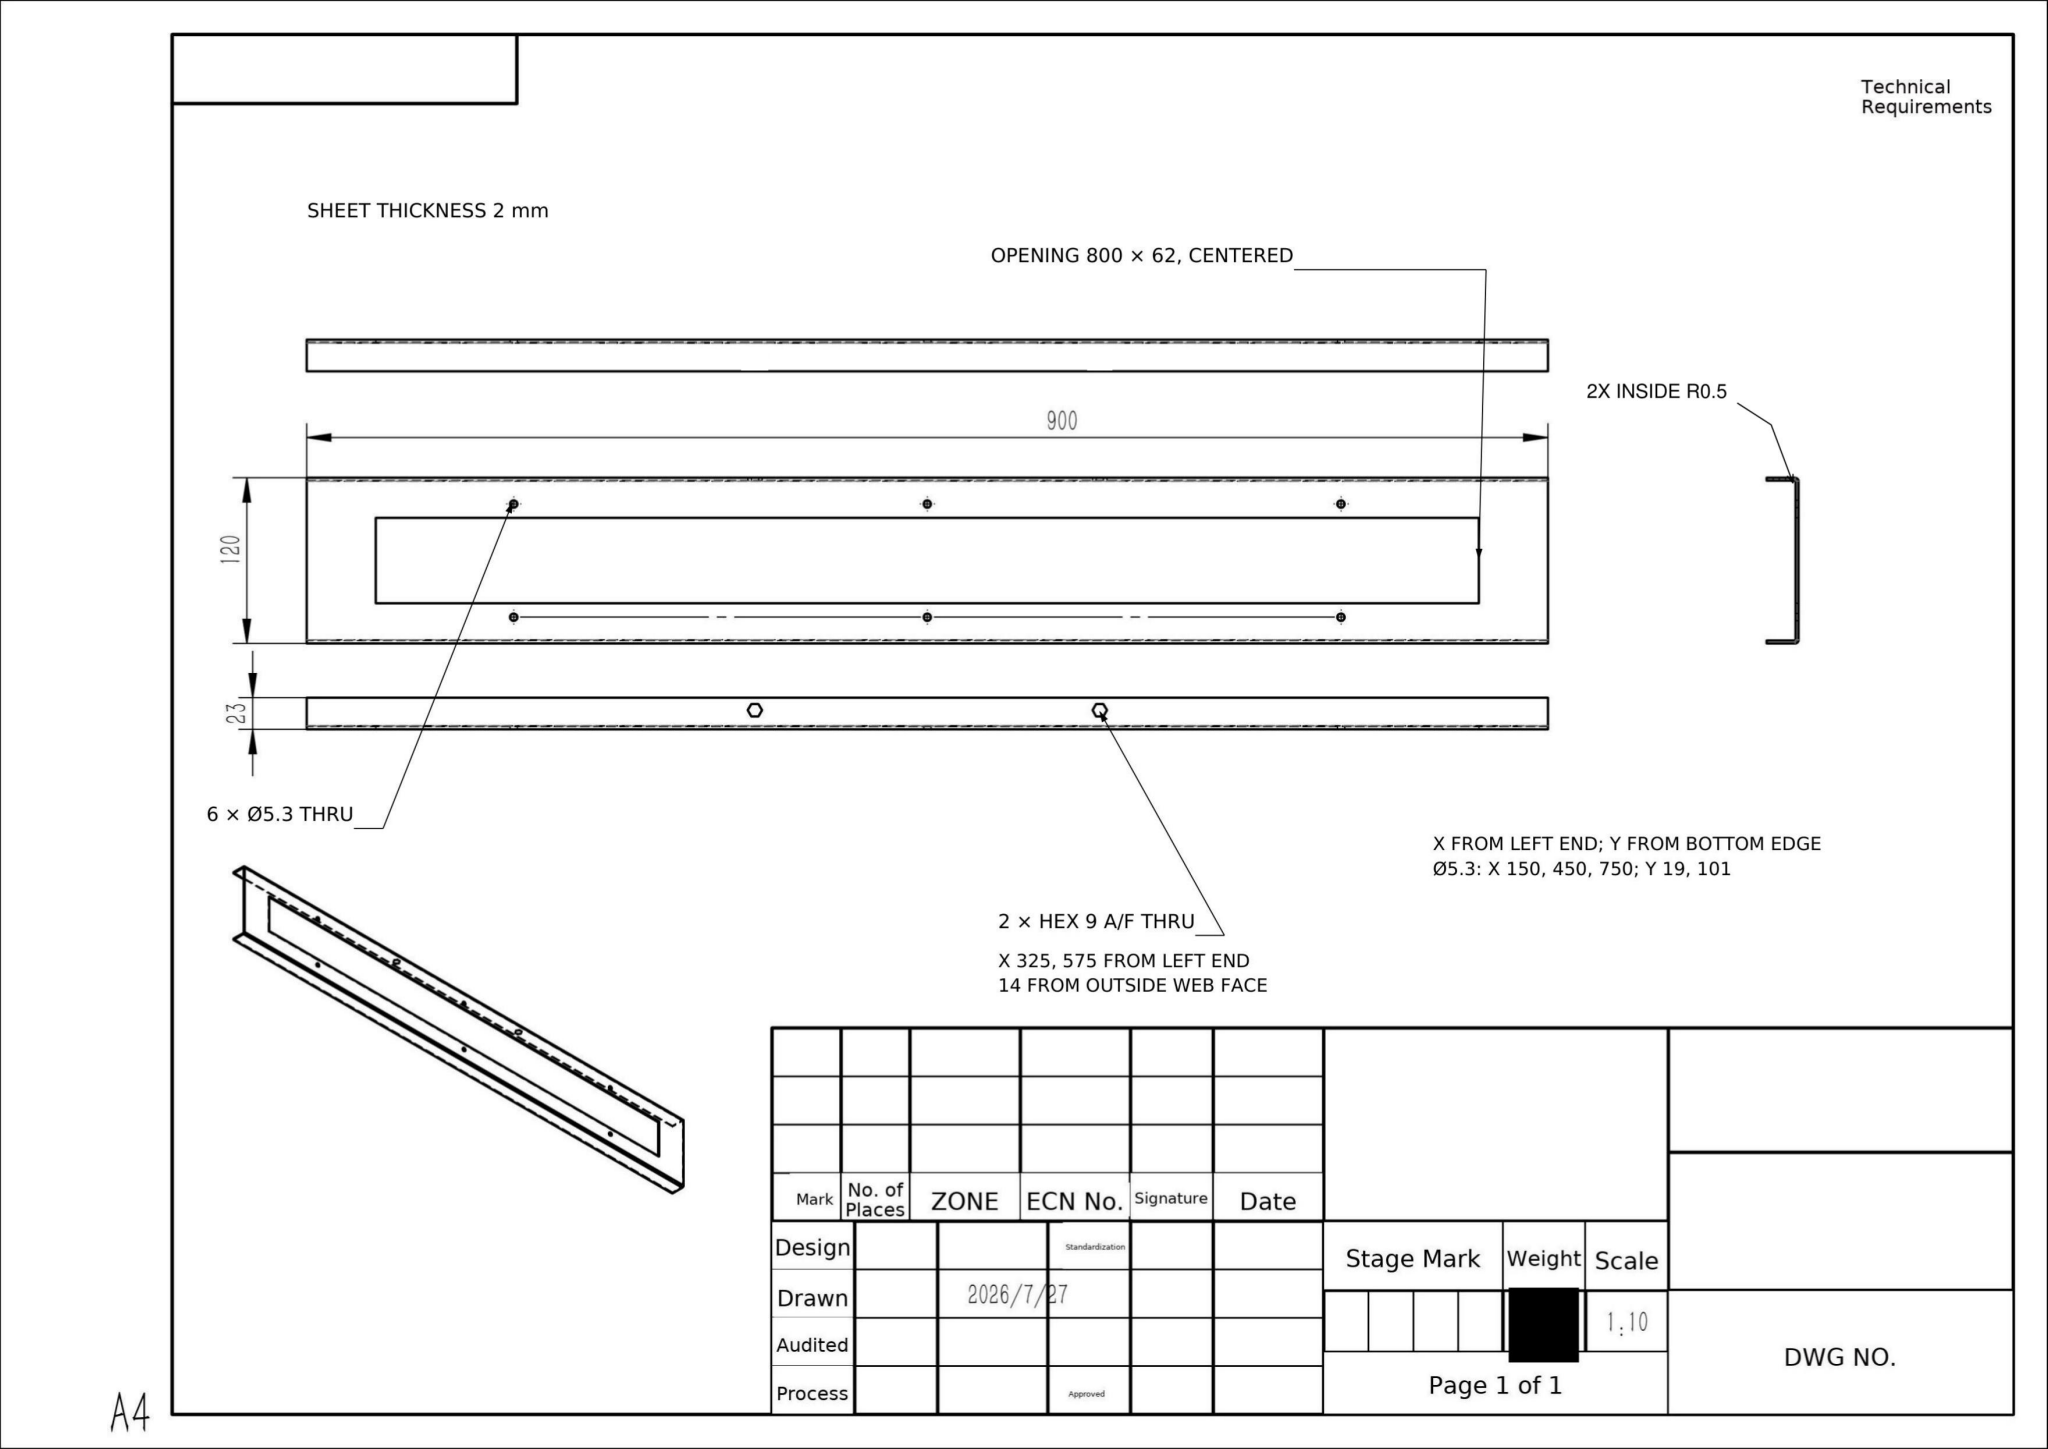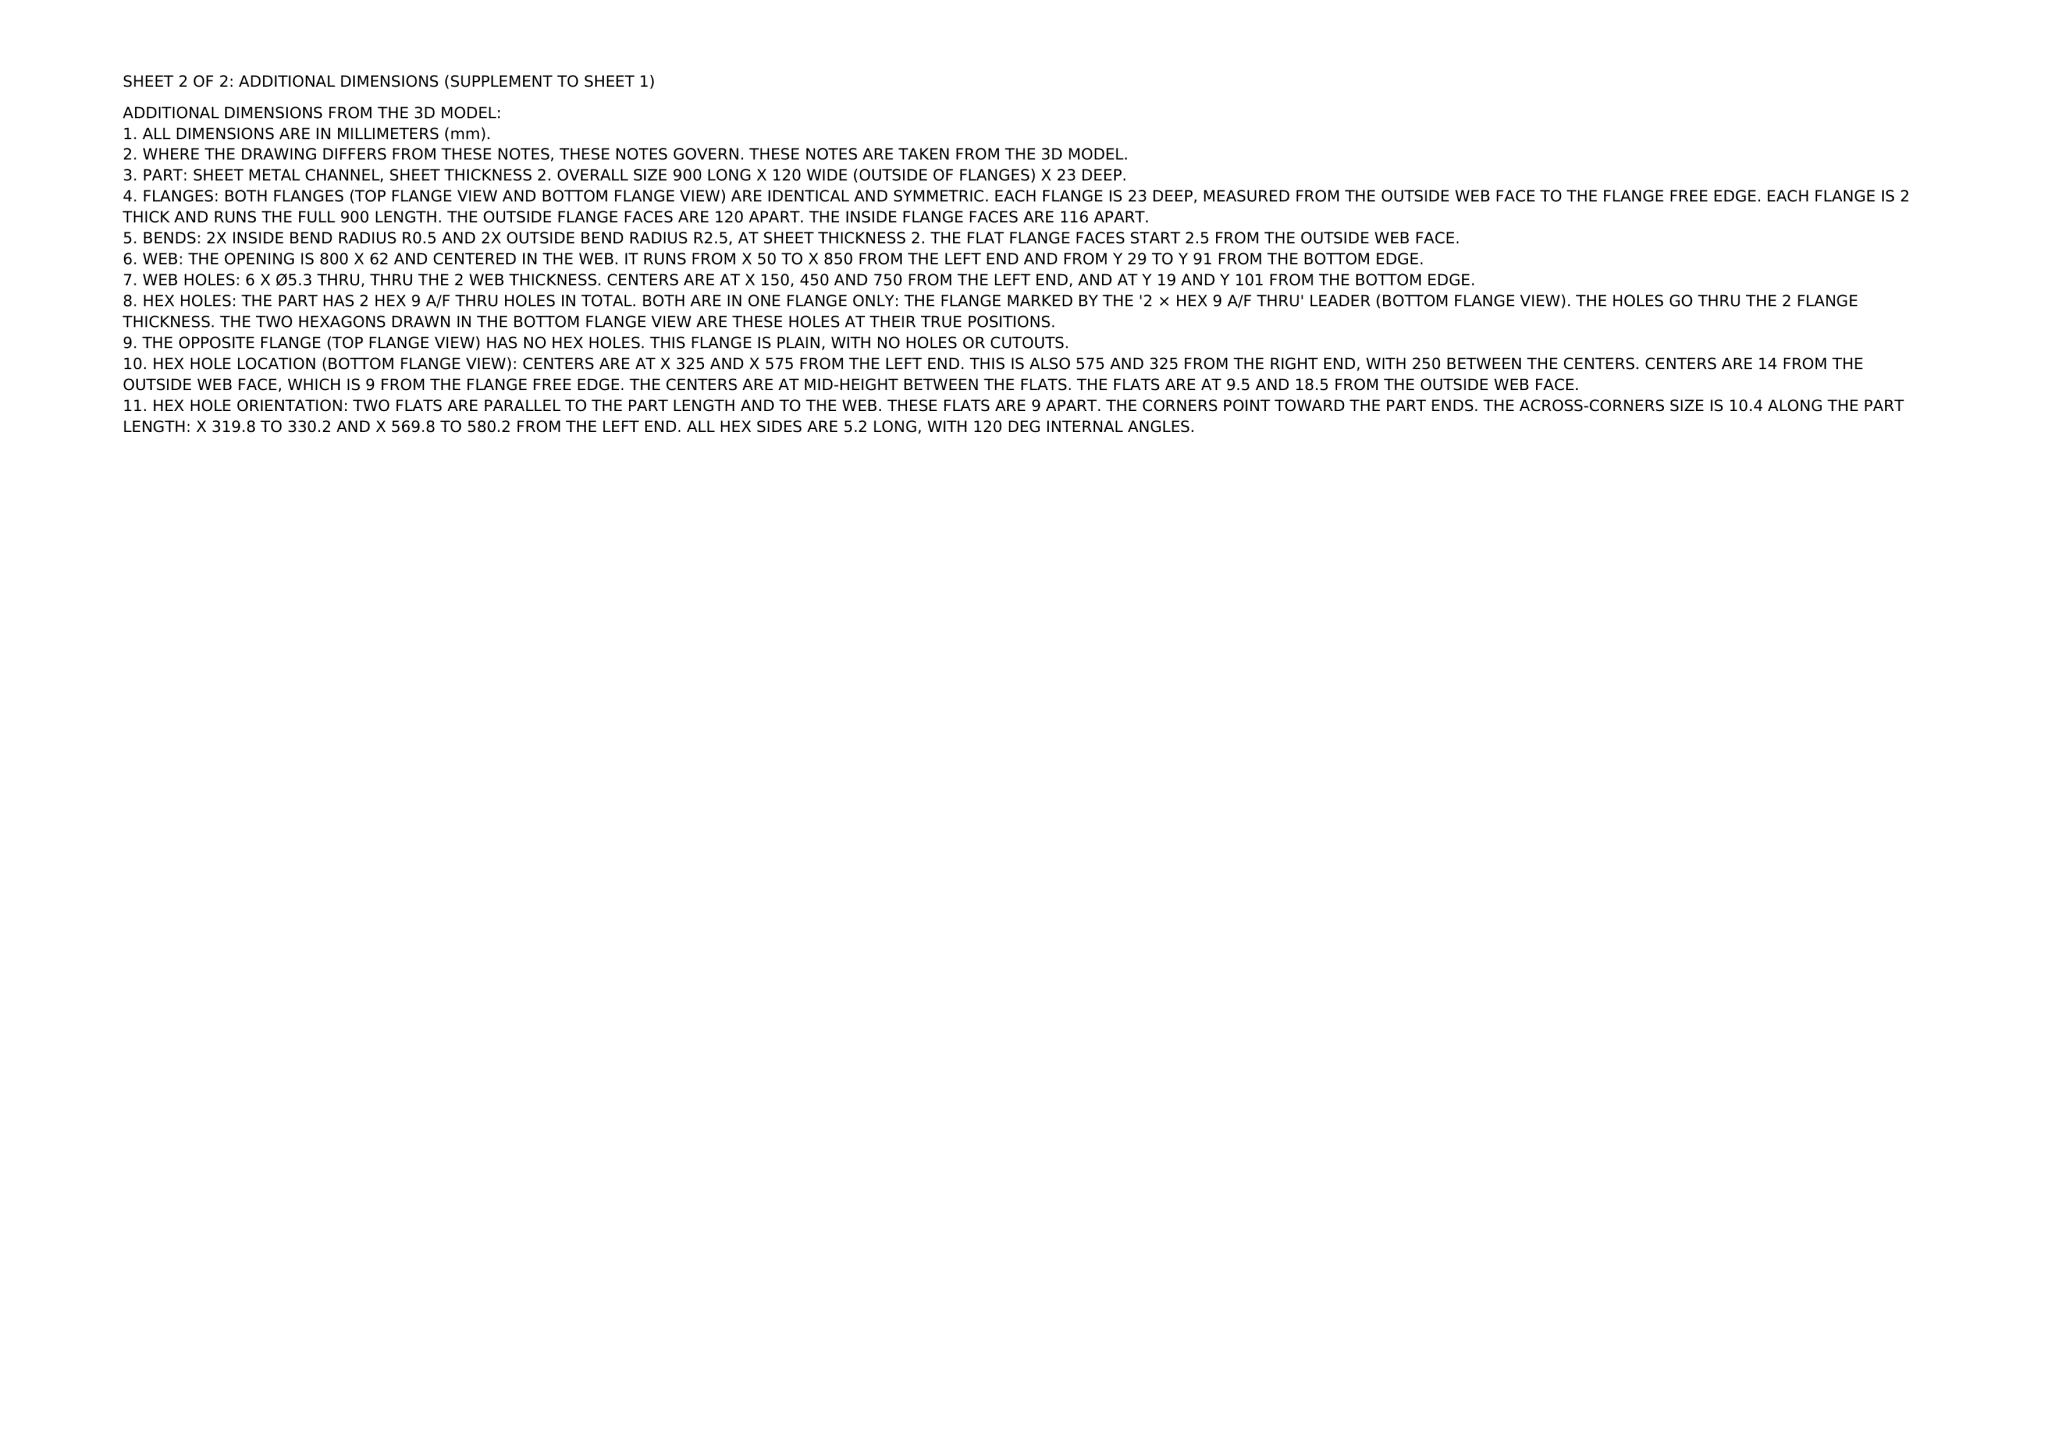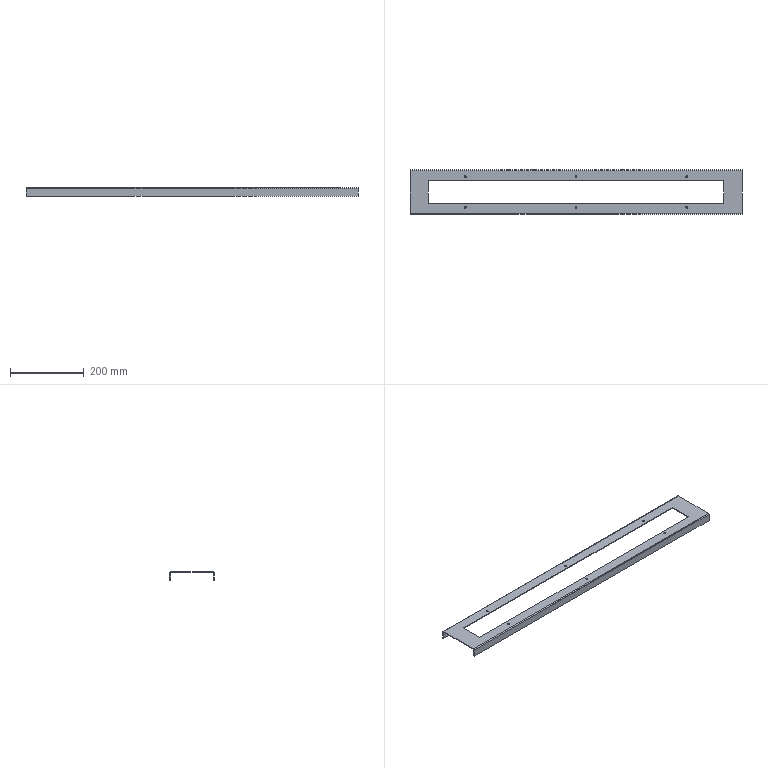Part | NX | mm | Rectangular Aperture Mounting Frame 900mm | 1 solid | 50 faces | box 900 x 120 x 23 mm | volume 189537 mm3 | plane 34 | cylinder 16 | commonest cylinder face diameters 5.3 x12 5 x2 1 x2